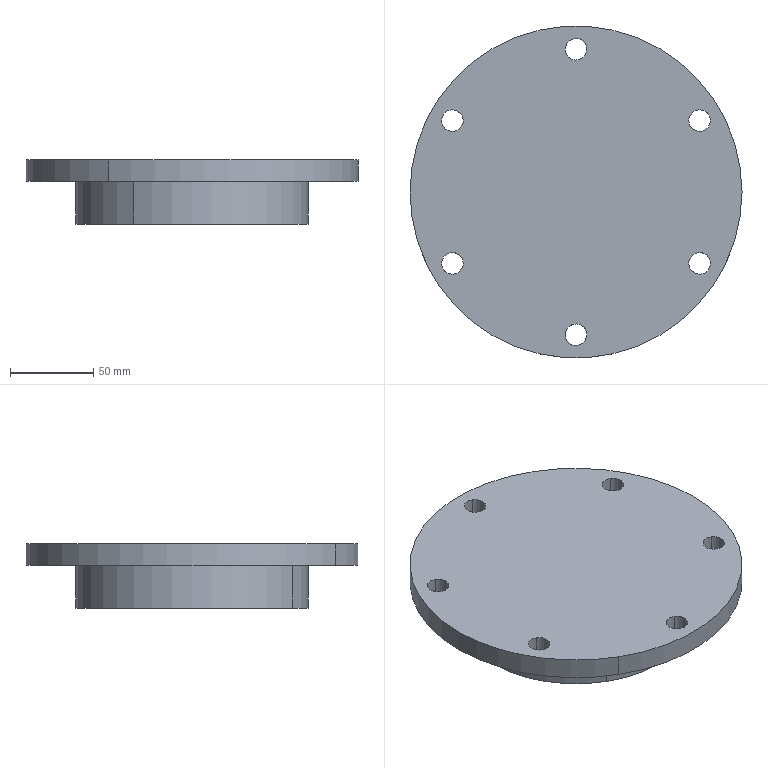Component | SolidWorks | PartAssemblyInLowerHousing-1_FlangeOnLowSpeedAxis1-1 | 1 solid | 22 faces | box 200 x 200 x 38.75 mm | volume 478948 mm3 | cylinder 16 | plane 4 | cone 2 | commonest cylinder face diameters 13 x12 200 x2 140 x2
build123d program:
from build123d import *

# Parameters (mm, degrees)
SKETCH2_R          = 6.5
CUT_EXTRUDE2_DEPTH = 147.634
CIRPATTERN1_COUNT  = 6
DRAFT1_ANGLE       = 2


with BuildPart() as part:
    # Sketch1 → Revolve1 (revolve)
    with BuildSketch(Plane.XY, mode=Mode.PRIVATE) as revolve1_sk:
        Polygon((0, 0), (13, 0), (13, 62), (38.75, 62), (38.75, 70), (13, 70), (13, 100), (0, 100), align=None)
    revolve(revolve1_sk.sketch.rotate(Axis((0, 0, 0), (1, 0, 0)), 90), axis=Axis((0, 0, 0), (1, 0, 0)))

    # Sketch2 → Cut-Extrude2 (cut, through all)
    with BuildSketch(Plane.ZY):
        with Locations((0, 86)):
            Circle(SKETCH2_R)
    cut_extrude2 = extrude(amount=-CUT_EXTRUDE2_DEPTH, mode=Mode.SUBTRACT)

    # CirPattern1: Cut-Extrude2 ×6 about axis
    cirpattern1_axis = Axis((0, 0, 0), (1, 0, 0))
    for i in range(1, CIRPATTERN1_COUNT):
        add(cut_extrude2.rotate(cirpattern1_axis, i * 360 / CIRPATTERN1_COUNT), mode=Mode.SUBTRACT)

    # Draft1
    draft1_faces = [part.faces().sort_by_distance(p)[0] for p in [
        (25.875, 0, -62),
    ]]
    draft(draft1_faces, Plane(origin=(13, 0, 0), x_dir=(0, 0, 1), z_dir=(1, 0, 0)), DRAFT1_ANGLE)


solid = part.part

# Placed as in the assembly
solid = solid.moved(Location((1140.83, 1268.591, 1836.217), (0, 90, 0)))
STEP:
#1=COLOUR_RGB('',0.7922,0.8196,0.9333);
#2=FILL_AREA_STYLE_COLOUR('',#1);
#3=FILL_AREA_STYLE('',(#2));
#4=SURFACE_STYLE_FILL_AREA(#3);
#5=SURFACE_SIDE_STYLE('',(#4));
#6=SURFACE_STYLE_USAGE(.BOTH.,#5);
#7=PRESENTATION_STYLE_ASSIGNMENT((#6));
#8=CARTESIAN_POINT('',(44.787,53.109,71.78));
#9=VERTEX_POINT('',#8);
#10=CARTESIAN_POINT('',(45.043,53.552,71.78));
#11=VERTEX_POINT('',#10);
#12=CARTESIAN_POINT('',(44.915,53.33,71.78));
#13=DIRECTION('',(0.,0.,1.));
#14=DIRECTION('',(0.5,0.866,0.));
#15=AXIS2_PLACEMENT_3D('',#12,#13,#14);
#16=CIRCLE('',#15,0.2559);
#17=EDGE_CURVE('',#9,#11,#16,.T.);
#18=ORIENTED_EDGE('',*,*,#17,.F.);
#19=CARTESIAN_POINT('',(44.787,53.109,72.292));
#20=VERTEX_POINT('',#19);
#21=CARTESIAN_POINT('',(44.787,53.109,70.766));
#22=DIRECTION('',(0.,0.,1.));
#23=VECTOR('',#22,39.37);
#24=LINE('',#21,#23);
#25=EDGE_CURVE('',#9,#20,#24,.T.);
#26=ORIENTED_EDGE('',*,*,#25,.T.);
#27=CARTESIAN_POINT('',(45.043,53.552,72.292));
#28=VERTEX_POINT('',#27);
#29=CARTESIAN_POINT('',(44.915,53.33,72.292));
#30=DIRECTION('',(0.,0.,1.));
#31=DIRECTION('',(1.,0.,0.));
#32=AXIS2_PLACEMENT_3D('',#29,#30,#31);
#33=CIRCLE('',#32,0.2559);
#34=EDGE_CURVE('',#20,#28,#33,.T.);
#35=ORIENTED_EDGE('',*,*,#34,.T.);
#36=CARTESIAN_POINT('',(45.043,53.552,70.766));
#37=DIRECTION('',(0.,0.,1.));
#38=VECTOR('',#37,39.37);
#39=LINE('',#36,#38);
#40=EDGE_CURVE('',#11,#28,#39,.T.);
#41=ORIENTED_EDGE('',*,*,#40,.F.);
#42=EDGE_LOOP('',(#18,#26,#35,#41));
#43=FACE_OUTER_BOUND('',#42,.T.);
#44=CARTESIAN_POINT('',(44.915,53.33,70.766));
#45=DIRECTION('',(0.,0.,1.));
#46=DIRECTION('',(0.5,0.866,0.));
#47=AXIS2_PLACEMENT_3D('',#44,#45,#46);
#48=CYLINDRICAL_SURFACE('',#47,0.2559);
#49=ADVANCED_FACE('',(#43),#48,.F.);
#50=CARTESIAN_POINT('',(47.719,51.416,71.78));
#51=VERTEX_POINT('',#50);
#52=CARTESIAN_POINT('',(47.975,51.859,71.78));
#53=VERTEX_POINT('',#52);
#54=CARTESIAN_POINT('',(47.847,51.637,71.78));
#55=DIRECTION('',(0.,0.,1.));
#56=DIRECTION('',(0.5,0.866,0.));
#57=AXIS2_PLACEMENT_3D('',#54,#55,#56);
#58=CIRCLE('',#57,0.2559);
#59=EDGE_CURVE('',#51,#53,#58,.T.);
#60=ORIENTED_EDGE('',*,*,#59,.F.);
#61=CARTESIAN_POINT('',(47.719,51.416,72.292));
#62=VERTEX_POINT('',#61);
#63=CARTESIAN_POINT('',(47.719,51.416,70.766));
#64=DIRECTION('',(0.,0.,1.));
#65=VECTOR('',#64,39.37);
#66=LINE('',#63,#65);
#67=EDGE_CURVE('',#51,#62,#66,.T.);
#68=ORIENTED_EDGE('',*,*,#67,.T.);
#69=CARTESIAN_POINT('',(47.975,51.859,72.292));
#70=VERTEX_POINT('',#69);
#71=CARTESIAN_POINT('',(47.847,51.637,72.292));
#72=DIRECTION('',(0.,0.,1.));
#73=DIRECTION('',(0.5,-0.866,0.));
#74=AXIS2_PLACEMENT_3D('',#71,#72,#73);
#75=CIRCLE('',#74,0.2559);
#76=EDGE_CURVE('',#62,#70,#75,.T.);
#77=ORIENTED_EDGE('',*,*,#76,.T.);
#78=CARTESIAN_POINT('',(47.975,51.859,70.766));
#79=DIRECTION('',(0.,0.,1.));
#80=VECTOR('',#79,39.37);
#81=LINE('',#78,#80);
#82=EDGE_CURVE('',#53,#70,#81,.T.);
#83=ORIENTED_EDGE('',*,*,#82,.F.);
#84=EDGE_LOOP('',(#60,#68,#77,#83));
#85=FACE_OUTER_BOUND('',#84,.T.);
#86=CARTESIAN_POINT('',(47.847,51.637,70.766));
#87=DIRECTION('',(0.,0.,1.));
#88=DIRECTION('',(0.5,0.866,0.));
#89=AXIS2_PLACEMENT_3D('',#86,#87,#88);
#90=CYLINDRICAL_SURFACE('',#89,0.2559);
#91=ADVANCED_FACE('',(#85),#90,.F.);
#92=CARTESIAN_POINT('',(47.719,48.03,71.78));
#93=VERTEX_POINT('',#92);
#94=CARTESIAN_POINT('',(47.975,48.473,71.78));
#95=VERTEX_POINT('',#94);
#96=CARTESIAN_POINT('',(47.847,48.252,71.78));
#97=DIRECTION('',(0.,0.,1.));
#98=DIRECTION('',(0.5,0.866,0.));
#99=AXIS2_PLACEMENT_3D('',#96,#97,#98);
#100=CIRCLE('',#99,0.2559);
#101=EDGE_CURVE('',#93,#95,#100,.T.);
#102=ORIENTED_EDGE('',*,*,#101,.F.);
#103=CARTESIAN_POINT('',(47.719,48.03,72.292));
#104=VERTEX_POINT('',#103);
#105=CARTESIAN_POINT('',(47.719,48.03,70.766));
#106=DIRECTION('',(0.,0.,1.));
#107=VECTOR('',#106,39.37);
#108=LINE('',#105,#107);
#109=EDGE_CURVE('',#93,#104,#108,.T.);
#110=ORIENTED_EDGE('',*,*,#109,.T.);
#111=CARTESIAN_POINT('',(47.975,48.473,72.292));
#112=VERTEX_POINT('',#111);
#113=CARTESIAN_POINT('',(47.847,48.252,72.292));
#114=DIRECTION('',(0.,0.,1.));
#115=DIRECTION('',(-0.5,-0.866,0.));
#116=AXIS2_PLACEMENT_3D('',#113,#114,#115);
#117=CIRCLE('',#116,0.2559);
#118=EDGE_CURVE('',#104,#112,#117,.T.);
#119=ORIENTED_EDGE('',*,*,#118,.T.);
#120=CARTESIAN_POINT('',(47.975,48.473,70.766));
#121=DIRECTION('',(0.,0.,1.));
#122=VECTOR('',#121,39.37);
#123=LINE('',#120,#122);
#124=EDGE_CURVE('',#95,#112,#123,.T.);
#125=ORIENTED_EDGE('',*,*,#124,.F.);
#126=EDGE_LOOP('',(#102,#110,#119,#125));
#127=FACE_OUTER_BOUND('',#126,.T.);
#128=CARTESIAN_POINT('',(47.847,48.252,70.766));
#129=DIRECTION('',(0.,0.,1.));
#130=DIRECTION('',(0.5,0.866,0.));
#131=AXIS2_PLACEMENT_3D('',#128,#129,#130);
#132=CYLINDRICAL_SURFACE('',#131,0.2559);
#133=ADVANCED_FACE('',(#127),#132,.F.);
#134=CARTESIAN_POINT('',(44.787,46.337,71.78));
#135=VERTEX_POINT('',#134);
#136=CARTESIAN_POINT('',(45.043,46.78,71.78));
#137=VERTEX_POINT('',#136);
#138=CARTESIAN_POINT('',(44.915,46.559,71.78));
#139=DIRECTION('',(0.,0.,1.));
#140=DIRECTION('',(0.5,0.866,0.));
#141=AXIS2_PLACEMENT_3D('',#138,#139,#140);
#142=CIRCLE('',#141,0.2559);
#143=EDGE_CURVE('',#135,#137,#142,.T.);
#144=ORIENTED_EDGE('',*,*,#143,.F.);
#145=CARTESIAN_POINT('',(44.787,46.337,72.292));
#146=VERTEX_POINT('',#145);
#147=CARTESIAN_POINT('',(44.787,46.337,70.766));
#148=DIRECTION('',(0.,0.,1.));
#149=VECTOR('',#148,39.37);
#150=LINE('',#147,#149);
#151=EDGE_CURVE('',#135,#146,#150,.T.);
#152=ORIENTED_EDGE('',*,*,#151,.T.);
#153=CARTESIAN_POINT('',(45.043,46.78,72.292));
#154=VERTEX_POINT('',#153);
#155=CARTESIAN_POINT('',(44.915,46.559,72.292));
#156=DIRECTION('',(0.,0.,1.));
#157=DIRECTION('',(-1.,0.,0.));
#158=AXIS2_PLACEMENT_3D('',#155,#156,#157);
#159=CIRCLE('',#158,0.2559);
#160=EDGE_CURVE('',#146,#154,#159,.T.);
#161=ORIENTED_EDGE('',*,*,#160,.T.);
#162=CARTESIAN_POINT('',(45.043,46.78,70.766));
#163=DIRECTION('',(0.,0.,1.));
#164=VECTOR('',#163,39.37);
#165=LINE('',#162,#164);
#166=EDGE_CURVE('',#137,#154,#165,.T.);
#167=ORIENTED_EDGE('',*,*,#166,.F.);
#168=EDGE_LOOP('',(#144,#152,#161,#167));
#169=FACE_OUTER_BOUND('',#168,.T.);
#170=CARTESIAN_POINT('',(44.915,46.559,70.766));
#171=DIRECTION('',(0.,0.,1.));
#172=DIRECTION('',(0.5,0.866,0.));
#173=AXIS2_PLACEMENT_3D('',#170,#171,#172);
#174=CYLINDRICAL_SURFACE('',#173,0.2559);
#175=ADVANCED_FACE('',(#169),#174,.F.);
#176=CARTESIAN_POINT('',(41.854,48.03,71.78));
#177=VERTEX_POINT('',#176);
#178=CARTESIAN_POINT('',(42.11,48.473,71.78));
#179=VERTEX_POINT('',#178);
#180=CARTESIAN_POINT('',(41.982,48.252,71.78));
#181=DIRECTION('',(0.,0.,1.));
#182=DIRECTION('',(0.5,0.866,0.));
#183=AXIS2_PLACEMENT_3D('',#180,#181,#182);
#184=CIRCLE('',#183,0.2559);
#185=EDGE_CURVE('',#177,#179,#184,.T.);
#186=ORIENTED_EDGE('',*,*,#185,.F.);
#187=CARTESIAN_POINT('',(41.854,48.03,72.292));
#188=VERTEX_POINT('',#187);
#189=CARTESIAN_POINT('',(41.854,48.03,70.766));
#190=DIRECTION('',(0.,0.,1.));
#191=VECTOR('',#190,39.37);
#192=LINE('',#189,#191);
#193=EDGE_CURVE('',#177,#188,#192,.T.);
#194=ORIENTED_EDGE('',*,*,#193,.T.);
#195=CARTESIAN_POINT('',(42.11,48.473,72.292));
#196=VERTEX_POINT('',#195);
#197=CARTESIAN_POINT('',(41.982,48.252,72.292));
#198=DIRECTION('',(0.,0.,1.));
#199=DIRECTION('',(-0.5,0.866,0.));
#200=AXIS2_PLACEMENT_3D('',#197,#198,#199);
#201=CIRCLE('',#200,0.2559);
#202=EDGE_CURVE('',#188,#196,#201,.T.);
#203=ORIENTED_EDGE('',*,*,#202,.T.);
#204=CARTESIAN_POINT('',(42.11,48.473,70.766));
#205=DIRECTION('',(0.,0.,1.));
#206=VECTOR('',#205,39.37);
#207=LINE('',#204,#206);
#208=EDGE_CURVE('',#179,#196,#207,.T.);
#209=ORIENTED_EDGE('',*,*,#208,.F.);
#210=EDGE_LOOP('',(#186,#194,#203,#209));
#211=FACE_OUTER_BOUND('',#210,.T.);
#212=CARTESIAN_POINT('',(41.982,48.252,70.766));
#213=DIRECTION('',(0.,0.,1.));
#214=DIRECTION('',(0.5,0.866,0.));
#215=AXIS2_PLACEMENT_3D('',#212,#213,#214);
#216=CYLINDRICAL_SURFACE('',#215,0.2559);
#217=ADVANCED_FACE('',(#211),#216,.F.);
#218=CARTESIAN_POINT('',(41.854,51.416,71.78));
#219=VERTEX_POINT('',#218);
#220=CARTESIAN_POINT('',(42.11,51.859,71.78));
#221=VERTEX_POINT('',#220);
#222=CARTESIAN_POINT('',(41.982,51.637,71.78));
#223=DIRECTION('',(0.,0.,1.));
#224=DIRECTION('',(0.5,0.866,0.));
#225=AXIS2_PLACEMENT_3D('',#222,#223,#224);
#226=CIRCLE('',#225,0.2559);
#227=EDGE_CURVE('',#219,#221,#226,.T.);
#228=ORIENTED_EDGE('',*,*,#227,.F.);
#229=CARTESIAN_POINT('',(41.854,51.416,72.292));
#230=VERTEX_POINT('',#229);
#231=CARTESIAN_POINT('',(41.854,51.416,70.766));
#232=DIRECTION('',(0.,0.,1.));
#233=VECTOR('',#232,39.37);
#234=LINE('',#231,#233);
#235=EDGE_CURVE('',#219,#230,#234,.T.);
#236=ORIENTED_EDGE('',*,*,#235,.T.);
#237=CARTESIAN_POINT('',(42.11,51.859,72.292));
#238=VERTEX_POINT('',#237);
#239=CARTESIAN_POINT('',(41.982,51.637,72.292));
#240=DIRECTION('',(0.,0.,1.));
#241=DIRECTION('',(0.5,0.866,0.));
#242=AXIS2_PLACEMENT_3D('',#239,#240,#241);
#243=CIRCLE('',#242,0.2559);
#244=EDGE_CURVE('',#230,#238,#243,.T.);
#245=ORIENTED_EDGE('',*,*,#244,.T.);
#246=CARTESIAN_POINT('',(42.11,51.859,70.766));
#247=DIRECTION('',(0.,0.,1.));
#248=VECTOR('',#247,39.37);
#249=LINE('',#246,#248);
#250=EDGE_CURVE('',#221,#238,#249,.T.);
#251=ORIENTED_EDGE('',*,*,#250,.F.);
#252=EDGE_LOOP('',(#228,#236,#245,#251));
#253=FACE_OUTER_BOUND('',#252,.T.);
#254=CARTESIAN_POINT('',(41.982,51.637,70.766));
#255=DIRECTION('',(0.,0.,1.));
#256=DIRECTION('',(0.5,0.866,0.));
#257=AXIS2_PLACEMENT_3D('',#254,#255,#256);
#258=CYLINDRICAL_SURFACE('',#257,0.2559);
#259=ADVANCED_FACE('',(#253),#258,.F.);
#260=CARTESIAN_POINT('',(46.883,53.354,71.78));
#261=VERTEX_POINT('',#260);
#262=CARTESIAN_POINT('',(42.946,46.535,71.78));
#263=VERTEX_POINT('',#262);
#264=CARTESIAN_POINT('',(44.915,49.945,71.78));
#265=DIRECTION('',(0.,0.,1.));
#266=DIRECTION('',(0.5,0.866,0.));
#267=AXIS2_PLACEMENT_3D('',#264,#265,#266);
#268=CIRCLE('',#267,3.937);
#269=EDGE_CURVE('',#261,#263,#268,.T.);
#270=ORIENTED_EDGE('',*,*,#269,.T.);
#271=CARTESIAN_POINT('',(42.946,46.535,72.292));
#272=VERTEX_POINT('',#271);
#273=CARTESIAN_POINT('',(42.946,46.535,72.292));
#274=DIRECTION('',(0.,0.,1.));
#275=VECTOR('',#274,39.37);
#276=LINE('',#273,#275);
#277=EDGE_CURVE('',#263,#272,#276,.T.);
#278=ORIENTED_EDGE('',*,*,#277,.T.);
#279=CARTESIAN_POINT('',(46.883,53.354,72.292));
#280=VERTEX_POINT('',#279);
#281=CARTESIAN_POINT('',(44.915,49.945,72.292));
#282=DIRECTION('',(0.,0.,1.));
#283=DIRECTION('',(0.5,0.866,0.));
#284=AXIS2_PLACEMENT_3D('',#281,#282,#283);
#285=CIRCLE('',#284,3.937);
#286=EDGE_CURVE('',#280,#272,#285,.T.);
#287=ORIENTED_EDGE('',*,*,#286,.F.);
#288=CARTESIAN_POINT('',(46.883,53.354,72.292));
#289=DIRECTION('',(0.,0.,1.));
#290=VECTOR('',#289,39.37);
#291=LINE('',#288,#290);
#292=EDGE_CURVE('',#261,#280,#291,.T.);
#293=ORIENTED_EDGE('',*,*,#292,.F.);
#294=EDGE_LOOP('',(#270,#278,#287,#293));
#295=FACE_OUTER_BOUND('',#294,.T.);
#296=CARTESIAN_POINT('',(44.915,49.945,72.292));
#297=DIRECTION('',(0.,0.,1.));
#298=DIRECTION('',(0.5,0.866,0.));
#299=AXIS2_PLACEMENT_3D('',#296,#297,#298);
#300=CYLINDRICAL_SURFACE('',#299,3.937);
#301=ADVANCED_FACE('',(#295),#300,.T.);
#302=CARTESIAN_POINT('',(46.293,52.331,70.766));
#303=VERTEX_POINT('',#302);
#304=CARTESIAN_POINT('',(43.537,47.558,70.766));
#305=VERTEX_POINT('',#304);
#306=CARTESIAN_POINT('',(44.915,49.945,70.766));
#307=DIRECTION('',(0.,0.,1.));
#308=DIRECTION('',(0.5,0.866,0.));
#309=AXIS2_PLACEMENT_3D('',#306,#307,#308);
#310=CIRCLE('',#309,2.756);
#311=EDGE_CURVE('',#303,#305,#310,.T.);
#312=ORIENTED_EDGE('',*,*,#311,.T.);
#313=CARTESIAN_POINT('',(43.537,47.558,71.78));
#314=VERTEX_POINT('',#313);
#315=CARTESIAN_POINT('',(43.537,47.558,72.292));
#316=DIRECTION('',(0.,0.,1.));
#317=VECTOR('',#316,39.37);
#318=LINE('',#315,#317);
#319=EDGE_CURVE('',#305,#314,#318,.T.);
#320=ORIENTED_EDGE('',*,*,#319,.T.);
#321=CARTESIAN_POINT('',(46.293,52.331,71.78));
#322=VERTEX_POINT('',#321);
#323=CARTESIAN_POINT('',(44.915,49.945,71.78));
#324=DIRECTION('',(0.,0.,1.));
#325=DIRECTION('',(0.5,0.866,0.));
#326=AXIS2_PLACEMENT_3D('',#323,#324,#325);
#327=CIRCLE('',#326,2.756);
#328=EDGE_CURVE('',#322,#314,#327,.T.);
#329=ORIENTED_EDGE('',*,*,#328,.F.);
#330=CARTESIAN_POINT('',(46.293,52.331,72.292));
#331=DIRECTION('',(0.,0.,1.));
#332=VECTOR('',#331,39.37);
#333=LINE('',#330,#332);
#334=EDGE_CURVE('',#303,#322,#333,.T.);
#335=ORIENTED_EDGE('',*,*,#334,.F.);
#336=EDGE_LOOP('',(#312,#320,#329,#335));
#337=FACE_OUTER_BOUND('',#336,.T.);
#338=CARTESIAN_POINT('',(44.915,49.945,72.292));
#339=DIRECTION('',(0.,0.,1.));
#340=DIRECTION('',(0.5,0.866,0.));
#341=AXIS2_PLACEMENT_3D('',#338,#339,#340);
#342=CYLINDRICAL_SURFACE('',#341,2.756);
#343=ADVANCED_FACE('',(#337),#342,.T.);
#344=CARTESIAN_POINT('',(46.135,52.058,71.78));
#345=VERTEX_POINT('',#344);
#346=CARTESIAN_POINT('',(43.694,47.831,71.78));
#347=VERTEX_POINT('',#346);
#348=CARTESIAN_POINT('',(44.915,49.945,71.78));
#349=DIRECTION('',(0.,0.,1.));
#350=DIRECTION('',(0.5,0.866,0.));
#351=AXIS2_PLACEMENT_3D('',#348,#349,#350);
#352=CIRCLE('',#351,2.441);
#353=EDGE_CURVE('',#345,#347,#352,.T.);
#354=ORIENTED_EDGE('',*,*,#353,.T.);
#355=CARTESIAN_POINT('',(43.676,47.8,70.766));
#356=VERTEX_POINT('',#355);
#357=CARTESIAN_POINT('',(43.694,47.831,71.78));
#358=DIRECTION('',(-0.01745,-0.03022,-0.9994));
#359=VECTOR('',#358,39.37);
#360=LINE('',#357,#359);
#361=EDGE_CURVE('',#347,#356,#360,.T.);
#362=ORIENTED_EDGE('',*,*,#361,.T.);
#363=CARTESIAN_POINT('',(46.153,52.089,70.766));
#364=VERTEX_POINT('',#363);
#365=CARTESIAN_POINT('',(44.915,49.945,70.766));
#366=DIRECTION('',(0.,0.,1.));
#367=DIRECTION('',(0.5,0.866,0.));
#368=AXIS2_PLACEMENT_3D('',#365,#366,#367);
#369=CIRCLE('',#368,2.476);
#370=EDGE_CURVE('',#364,#356,#369,.T.);
#371=ORIENTED_EDGE('',*,*,#370,.F.);
#372=CARTESIAN_POINT('',(46.135,52.058,71.78));
#373=DIRECTION('',(0.01745,0.03022,-0.9994));
#374=VECTOR('',#373,39.37);
#375=LINE('',#372,#374);
#376=EDGE_CURVE('',#345,#364,#375,.T.);
#377=ORIENTED_EDGE('',*,*,#376,.F.);
#378=EDGE_LOOP('',(#354,#362,#371,#377));
#379=FACE_OUTER_BOUND('',#378,.T.);
#380=CARTESIAN_POINT('',(44.915,49.945,71.78));
#381=DIRECTION('',(0.,0.,-1.));
#382=DIRECTION('',(0.5,0.866,0.));
#383=AXIS2_PLACEMENT_3D('',#380,#381,#382);
#384=CONICAL_SURFACE('',#383,2.441,0.03491);
#385=ADVANCED_FACE('',(#379),#384,.F.);
#386=CARTESIAN_POINT('',(44.915,53.33,72.292));
#387=DIRECTION('',(0.,0.,1.));
#388=DIRECTION('',(1.,0.,0.));
#389=AXIS2_PLACEMENT_3D('',#386,#387,#388);
#390=CIRCLE('',#389,0.2559);
#391=EDGE_CURVE('',#28,#20,#390,.T.);
#392=ORIENTED_EDGE('',*,*,#391,.F.);
#393=ORIENTED_EDGE('',*,*,#34,.F.);
#394=EDGE_LOOP('',(#392,#393));
#395=FACE_BOUND('',#394,.T.);
#396=CARTESIAN_POINT('',(47.847,51.637,72.292));
#397=DIRECTION('',(0.,0.,1.));
#398=DIRECTION('',(0.5,-0.866,0.));
#399=AXIS2_PLACEMENT_3D('',#396,#397,#398);
#400=CIRCLE('',#399,0.2559);
#401=EDGE_CURVE('',#70,#62,#400,.T.);
#402=ORIENTED_EDGE('',*,*,#401,.F.);
#403=ORIENTED_EDGE('',*,*,#76,.F.);
#404=EDGE_LOOP('',(#402,#403));
#405=FACE_BOUND('',#404,.T.);
#406=CARTESIAN_POINT('',(47.847,48.252,72.292));
#407=DIRECTION('',(0.,0.,1.));
#408=DIRECTION('',(-0.5,-0.866,0.));
#409=AXIS2_PLACEMENT_3D('',#406,#407,#408);
#410=CIRCLE('',#409,0.2559);
#411=EDGE_CURVE('',#112,#104,#410,.T.);
#412=ORIENTED_EDGE('',*,*,#411,.F.);
#413=ORIENTED_EDGE('',*,*,#118,.F.);
#414=EDGE_LOOP('',(#412,#413));
#415=FACE_BOUND('',#414,.T.);
#416=CARTESIAN_POINT('',(44.915,46.559,72.292));
#417=DIRECTION('',(0.,0.,1.));
#418=DIRECTION('',(-1.,0.,0.));
#419=AXIS2_PLACEMENT_3D('',#416,#417,#418);
#420=CIRCLE('',#419,0.2559);
#421=EDGE_CURVE('',#154,#146,#420,.T.);
#422=ORIENTED_EDGE('',*,*,#421,.F.);
#423=ORIENTED_EDGE('',*,*,#160,.F.);
#424=EDGE_LOOP('',(#422,#423));
#425=FACE_BOUND('',#424,.T.);
#426=CARTESIAN_POINT('',(41.982,48.252,72.292));
#427=DIRECTION('',(0.,0.,1.));
#428=DIRECTION('',(-0.5,0.866,0.));
#429=AXIS2_PLACEMENT_3D('',#426,#427,#428);
#430=CIRCLE('',#429,0.2559);
#431=EDGE_CURVE('',#196,#188,#430,.T.);
#432=ORIENTED_EDGE('',*,*,#431,.F.);
#433=ORIENTED_EDGE('',*,*,#202,.F.);
#434=EDGE_LOOP('',(#432,#433));
#435=FACE_BOUND('',#434,.T.);
#436=CARTESIAN_POINT('',(41.982,51.637,72.292));
#437=DIRECTION('',(0.,0.,1.));
#438=DIRECTION('',(0.5,0.866,0.));
#439=AXIS2_PLACEMENT_3D('',#436,#437,#438);
#440=CIRCLE('',#439,0.2559);
#441=EDGE_CURVE('',#238,#230,#440,.T.);
#442=ORIENTED_EDGE('',*,*,#441,.F.);
#443=ORIENTED_EDGE('',*,*,#244,.F.);
#444=EDGE_LOOP('',(#442,#443));
#445=FACE_BOUND('',#444,.T.);
#446=ORIENTED_EDGE('',*,*,#286,.T.);
#447=CARTESIAN_POINT('',(44.915,49.945,72.292));
#448=DIRECTION('',(0.,0.,1.));
#449=DIRECTION('',(0.5,0.866,0.));
#450=AXIS2_PLACEMENT_3D('',#447,#448,#449);
#451=CIRCLE('',#450,3.937);
#452=EDGE_CURVE('',#272,#280,#451,.T.);
#453=ORIENTED_EDGE('',*,*,#452,.T.);
#454=EDGE_LOOP('',(#446,#453));
#455=FACE_OUTER_BOUND('',#454,.T.);
#456=CARTESIAN_POINT('',(41.505,51.913,72.292));
#457=DIRECTION('',(0.,0.,-1.));
#458=DIRECTION('',(-0.5,-0.866,0.));
#459=AXIS2_PLACEMENT_3D('',#456,#457,#458);
#460=PLANE('',#459);
#461=ADVANCED_FACE('',(#395,#405,#415,#425,#435,#445,#455),#460,.F.);
#462=ORIENTED_EDGE('',*,*,#353,.F.);
#463=CARTESIAN_POINT('',(44.915,49.945,71.78));
#464=DIRECTION('',(0.,0.,1.));
#465=DIRECTION('',(0.5,0.866,0.));
#466=AXIS2_PLACEMENT_3D('',#463,#464,#465);
#467=CIRCLE('',#466,2.441);
#468=EDGE_CURVE('',#347,#345,#467,.T.);
#469=ORIENTED_EDGE('',*,*,#468,.F.);
#470=EDGE_LOOP('',(#462,#469));
#471=FACE_OUTER_BOUND('',#470,.T.);
#472=CARTESIAN_POINT('',(44.915,49.945,71.78));
#473=DIRECTION('',(0.,0.,1.));
#474=DIRECTION('',(0.5,0.866,0.));
#475=AXIS2_PLACEMENT_3D('',#472,#473,#474);
#476=PLANE('',#475);
#477=ADVANCED_FACE('',(#471),#476,.F.);
#478=ORIENTED_EDGE('',*,*,#361,.F.);
#479=ORIENTED_EDGE('',*,*,#468,.T.);
#480=ORIENTED_EDGE('',*,*,#376,.T.);
#481=CARTESIAN_POINT('',(44.915,49.945,70.766));
#482=DIRECTION('',(0.,0.,1.));
#483=DIRECTION('',(0.5,0.866,0.));
#484=AXIS2_PLACEMENT_3D('',#481,#482,#483);
#485=CIRCLE('',#484,2.476);
#486=EDGE_CURVE('',#356,#364,#485,.T.);
#487=ORIENTED_EDGE('',*,*,#486,.F.);
#488=EDGE_LOOP('',(#478,#479,#480,#487));
#489=FACE_OUTER_BOUND('',#488,.T.);
#490=CARTESIAN_POINT('',(44.915,49.945,71.78));
#491=DIRECTION('',(0.,0.,-1.));
#492=DIRECTION('',(0.5,0.866,0.));
#493=AXIS2_PLACEMENT_3D('',#490,#491,#492);
#494=CONICAL_SURFACE('',#493,2.441,0.03491);
#495=ADVANCED_FACE('',(#489),#494,.F.);
#496=ORIENTED_EDGE('',*,*,#311,.F.);
#497=CARTESIAN_POINT('',(44.915,49.945,70.766));
#498=DIRECTION('',(0.,0.,1.));
#499=DIRECTION('',(0.5,0.866,0.));
#500=AXIS2_PLACEMENT_3D('',#497,#498,#499);
#501=CIRCLE('',#500,2.756);
#502=EDGE_CURVE('',#305,#303,#501,.T.);
#503=ORIENTED_EDGE('',*,*,#502,.F.);
#504=EDGE_LOOP('',(#496,#503));
#505=FACE_OUTER_BOUND('',#504,.T.);
#506=ORIENTED_EDGE('',*,*,#370,.T.);
#507=ORIENTED_EDGE('',*,*,#486,.T.);
#508=EDGE_LOOP('',(#506,#507));
#509=FACE_BOUND('',#508,.T.);
#510=CARTESIAN_POINT('',(42.801,51.165,70.766));
#511=DIRECTION('',(0.,0.,1.));
#512=DIRECTION('',(0.5,0.866,0.));
#513=AXIS2_PLACEMENT_3D('',#510,#511,#512);
#514=PLANE('',#513);
#515=ADVANCED_FACE('',(#505,#509),#514,.F.);
#516=ORIENTED_EDGE('',*,*,#319,.F.);
#517=ORIENTED_EDGE('',*,*,#502,.T.);
#518=ORIENTED_EDGE('',*,*,#334,.T.);
#519=CARTESIAN_POINT('',(44.915,49.945,71.78));
#520=DIRECTION('',(0.,0.,1.));
#521=DIRECTION('',(0.5,0.866,0.));
#522=AXIS2_PLACEMENT_3D('',#519,#520,#521);
#523=CIRCLE('',#522,2.756);
#524=EDGE_CURVE('',#314,#322,#523,.T.);
#525=ORIENTED_EDGE('',*,*,#524,.F.);
#526=EDGE_LOOP('',(#516,#517,#518,#525));
#527=FACE_OUTER_BOUND('',#526,.T.);
#528=CARTESIAN_POINT('',(44.915,49.945,72.292));
#529=DIRECTION('',(0.,0.,1.));
#530=DIRECTION('',(0.5,0.866,0.));
#531=AXIS2_PLACEMENT_3D('',#528,#529,#530);
#532=CYLINDRICAL_SURFACE('',#531,2.756);
#533=ADVANCED_FACE('',(#527),#532,.T.);
#534=CARTESIAN_POINT('',(44.915,53.33,71.78));
#535=DIRECTION('',(0.,0.,1.));
#536=DIRECTION('',(0.5,0.866,0.));
#537=AXIS2_PLACEMENT_3D('',#534,#535,#536);
#538=CIRCLE('',#537,0.2559);
#539=EDGE_CURVE('',#11,#9,#538,.T.);
#540=ORIENTED_EDGE('',*,*,#539,.T.);
#541=ORIENTED_EDGE('',*,*,#17,.T.);
#542=EDGE_LOOP('',(#540,#541));
#543=FACE_BOUND('',#542,.T.);
#544=CARTESIAN_POINT('',(47.847,51.637,71.78));
#545=DIRECTION('',(0.,0.,1.));
#546=DIRECTION('',(0.5,0.866,0.));
#547=AXIS2_PLACEMENT_3D('',#544,#545,#546);
#548=CIRCLE('',#547,0.2559);
#549=EDGE_CURVE('',#53,#51,#548,.T.);
#550=ORIENTED_EDGE('',*,*,#549,.T.);
#551=ORIENTED_EDGE('',*,*,#59,.T.);
#552=EDGE_LOOP('',(#550,#551));
#553=FACE_BOUND('',#552,.T.);
#554=CARTESIAN_POINT('',(47.847,48.252,71.78));
#555=DIRECTION('',(0.,0.,1.));
#556=DIRECTION('',(0.5,0.866,0.));
#557=AXIS2_PLACEMENT_3D('',#554,#555,#556);
#558=CIRCLE('',#557,0.2559);
#559=EDGE_CURVE('',#95,#93,#558,.T.);
#560=ORIENTED_EDGE('',*,*,#559,.T.);
#561=ORIENTED_EDGE('',*,*,#101,.T.);
#562=EDGE_LOOP('',(#560,#561));
#563=FACE_BOUND('',#562,.T.);
#564=CARTESIAN_POINT('',(44.915,46.559,71.78));
#565=DIRECTION('',(0.,0.,1.));
#566=DIRECTION('',(0.5,0.866,0.));
#567=AXIS2_PLACEMENT_3D('',#564,#565,#566);
#568=CIRCLE('',#567,0.2559);
#569=EDGE_CURVE('',#137,#135,#568,.T.);
#570=ORIENTED_EDGE('',*,*,#569,.T.);
#571=ORIENTED_EDGE('',*,*,#143,.T.);
#572=EDGE_LOOP('',(#570,#571));
#573=FACE_BOUND('',#572,.T.);
#574=CARTESIAN_POINT('',(41.982,48.252,71.78));
#575=DIRECTION('',(0.,0.,1.));
#576=DIRECTION('',(0.5,0.866,0.));
#577=AXIS2_PLACEMENT_3D('',#574,#575,#576);
#578=CIRCLE('',#577,0.2559);
#579=EDGE_CURVE('',#179,#177,#578,.T.);
#580=ORIENTED_EDGE('',*,*,#579,.T.);
#581=ORIENTED_EDGE('',*,*,#185,.T.);
#582=EDGE_LOOP('',(#580,#581));
#583=FACE_BOUND('',#582,.T.);
#584=CARTESIAN_POINT('',(41.982,51.637,71.78));
#585=DIRECTION('',(0.,0.,1.));
#586=DIRECTION('',(0.5,0.866,0.));
#587=AXIS2_PLACEMENT_3D('',#584,#585,#586);
#588=CIRCLE('',#587,0.2559);
#589=EDGE_CURVE('',#221,#219,#588,.T.);
#590=ORIENTED_EDGE('',*,*,#589,.T.);
#591=ORIENTED_EDGE('',*,*,#227,.T.);
#592=EDGE_LOOP('',(#590,#591));
#593=FACE_BOUND('',#592,.T.);
#594=ORIENTED_EDGE('',*,*,#269,.F.);
#595=CARTESIAN_POINT('',(44.915,49.945,71.78));
#596=DIRECTION('',(0.,0.,1.));
#597=DIRECTION('',(0.5,0.866,0.));
#598=AXIS2_PLACEMENT_3D('',#595,#596,#597);
#599=CIRCLE('',#598,3.937);
#600=EDGE_CURVE('',#263,#261,#599,.T.);
#601=ORIENTED_EDGE('',*,*,#600,.F.);
#602=EDGE_LOOP('',(#594,#601));
#603=FACE_OUTER_BOUND('',#602,.T.);
#604=ORIENTED_EDGE('',*,*,#328,.T.);
#605=ORIENTED_EDGE('',*,*,#524,.T.);
#606=EDGE_LOOP('',(#604,#605));
#607=FACE_BOUND('',#606,.T.);
#608=CARTESIAN_POINT('',(42.528,51.322,71.78));
#609=DIRECTION('',(0.,0.,1.));
#610=DIRECTION('',(0.5,0.866,0.));
#611=AXIS2_PLACEMENT_3D('',#608,#609,#610);
#612=PLANE('',#611);
#613=ADVANCED_FACE('',(#543,#553,#563,#573,#583,#593,#603,#607),#612,.F.);
#614=ORIENTED_EDGE('',*,*,#277,.F.);
#615=ORIENTED_EDGE('',*,*,#600,.T.);
#616=ORIENTED_EDGE('',*,*,#292,.T.);
#617=ORIENTED_EDGE('',*,*,#452,.F.);
#618=EDGE_LOOP('',(#614,#615,#616,#617));
#619=FACE_OUTER_BOUND('',#618,.T.);
#620=CARTESIAN_POINT('',(44.915,49.945,72.292));
#621=DIRECTION('',(0.,0.,1.));
#622=DIRECTION('',(0.5,0.866,0.));
#623=AXIS2_PLACEMENT_3D('',#620,#621,#622);
#624=CYLINDRICAL_SURFACE('',#623,3.937);
#625=ADVANCED_FACE('',(#619),#624,.T.);
#626=ORIENTED_EDGE('',*,*,#235,.F.);
#627=ORIENTED_EDGE('',*,*,#589,.F.);
#628=ORIENTED_EDGE('',*,*,#250,.T.);
#629=ORIENTED_EDGE('',*,*,#441,.T.);
#630=EDGE_LOOP('',(#626,#627,#628,#629));
#631=FACE_OUTER_BOUND('',#630,.T.);
#632=CARTESIAN_POINT('',(41.982,51.637,70.766));
#633=DIRECTION('',(0.,0.,1.));
#634=DIRECTION('',(0.5,0.866,0.));
#635=AXIS2_PLACEMENT_3D('',#632,#633,#634);
#636=CYLINDRICAL_SURFACE('',#635,0.2559);
#637=ADVANCED_FACE('',(#631),#636,.F.);
#638=ORIENTED_EDGE('',*,*,#193,.F.);
#639=ORIENTED_EDGE('',*,*,#579,.F.);
#640=ORIENTED_EDGE('',*,*,#208,.T.);
#641=ORIENTED_EDGE('',*,*,#431,.T.);
#642=EDGE_LOOP('',(#638,#639,#640,#641));
#643=FACE_OUTER_BOUND('',#642,.T.);
#644=CARTESIAN_POINT('',(41.982,48.252,70.766));
#645=DIRECTION('',(0.,0.,1.));
#646=DIRECTION('',(0.5,0.866,0.));
#647=AXIS2_PLACEMENT_3D('',#644,#645,#646);
#648=CYLINDRICAL_SURFACE('',#647,0.2559);
#649=ADVANCED_FACE('',(#643),#648,.F.);
#650=ORIENTED_EDGE('',*,*,#151,.F.);
#651=ORIENTED_EDGE('',*,*,#569,.F.);
#652=ORIENTED_EDGE('',*,*,#166,.T.);
#653=ORIENTED_EDGE('',*,*,#421,.T.);
#654=EDGE_LOOP('',(#650,#651,#652,#653));
#655=FACE_OUTER_BOUND('',#654,.T.);
#656=CARTESIAN_POINT('',(44.915,46.559,70.766));
#657=DIRECTION('',(0.,0.,1.));
#658=DIRECTION('',(0.5,0.866,0.));
#659=AXIS2_PLACEMENT_3D('',#656,#657,#658);
#660=CYLINDRICAL_SURFACE('',#659,0.2559);
#661=ADVANCED_FACE('',(#655),#660,.F.);
#662=ORIENTED_EDGE('',*,*,#109,.F.);
#663=ORIENTED_EDGE('',*,*,#559,.F.);
#664=ORIENTED_EDGE('',*,*,#124,.T.);
#665=ORIENTED_EDGE('',*,*,#411,.T.);
#666=EDGE_LOOP('',(#662,#663,#664,#665));
#667=FACE_OUTER_BOUND('',#666,.T.);
#668=CARTESIAN_POINT('',(47.847,48.252,70.766));
#669=DIRECTION('',(0.,0.,1.));
#670=DIRECTION('',(0.5,0.866,0.));
#671=AXIS2_PLACEMENT_3D('',#668,#669,#670);
#672=CYLINDRICAL_SURFACE('',#671,0.2559);
#673=ADVANCED_FACE('',(#667),#672,.F.);
#674=ORIENTED_EDGE('',*,*,#67,.F.);
#675=ORIENTED_EDGE('',*,*,#549,.F.);
#676=ORIENTED_EDGE('',*,*,#82,.T.);
#677=ORIENTED_EDGE('',*,*,#401,.T.);
#678=EDGE_LOOP('',(#674,#675,#676,#677));
#679=FACE_OUTER_BOUND('',#678,.T.);
#680=CARTESIAN_POINT('',(47.847,51.637,70.766));
#681=DIRECTION('',(0.,0.,1.));
#682=DIRECTION('',(0.5,0.866,0.));
#683=AXIS2_PLACEMENT_3D('',#680,#681,#682);
#684=CYLINDRICAL_SURFACE('',#683,0.2559);
#685=ADVANCED_FACE('',(#679),#684,.F.);
#686=ORIENTED_EDGE('',*,*,#25,.F.);
#687=ORIENTED_EDGE('',*,*,#539,.F.);
#688=ORIENTED_EDGE('',*,*,#40,.T.);
#689=ORIENTED_EDGE('',*,*,#391,.T.);
#690=EDGE_LOOP('',(#686,#687,#688,#689));
#691=FACE_OUTER_BOUND('',#690,.T.);
#692=CARTESIAN_POINT('',(44.915,53.33,70.766));
#693=DIRECTION('',(0.,0.,1.));
#694=DIRECTION('',(0.5,0.866,0.));
#695=AXIS2_PLACEMENT_3D('',#692,#693,#694);
#696=CYLINDRICAL_SURFACE('',#695,0.2559);
#697=ADVANCED_FACE('',(#691),#696,.F.);
#698=CLOSED_SHELL('',(#49,#91,#133,#175,#217,#259,#301,#343,#385,#461,#477,#495,#515,#533,#613,#625,#637,#649,#661,#673,#685,#697));
#699=MANIFOLD_SOLID_BREP('',#698);
#700=STYLED_ITEM('',(#7),#699);
#701=(LENGTH_UNIT()NAMED_UNIT(*)SI_UNIT($,.METRE.));
#702=LENGTH_MEASURE_WITH_UNIT(LENGTH_MEASURE(0.0254),#701);
#703=DIMENSIONAL_EXPONENTS(1.,0.,0.,0.,0.,0.,0.);
#704=(CONVERSION_BASED_UNIT('',#702)LENGTH_UNIT()NAMED_UNIT(#703));
#705=UNCERTAINTY_MEASURE_WITH_UNIT(LENGTH_MEASURE(0.00001),#704,'','');
#706=(NAMED_UNIT(*)PLANE_ANGLE_UNIT()SI_UNIT($,.RADIAN.));
#707=(NAMED_UNIT(*)SI_UNIT($,.STERADIAN.)SOLID_ANGLE_UNIT());
#708=(GEOMETRIC_REPRESENTATION_CONTEXT(3)GLOBAL_UNCERTAINTY_ASSIGNED_CONTEXT((#705))GLOBAL_UNIT_ASSIGNED_CONTEXT((#704,#706,#707))REPRESENTATION_CONTEXT('',''));
#709=MECHANICAL_DESIGN_GEOMETRIC_PRESENTATION_REPRESENTATION('',(#700),#708);
#710=PRESENTATION_LAYER_ASSIGNMENT('','',(#700));
#711=CARTESIAN_POINT('',(0.,0.,0.));
#712=DIRECTION('',(0.,0.,1.));
#713=DIRECTION('',(1.,0.,0.));
#714=AXIS2_PLACEMENT_3D('',#711,#712,#713);
#715=(LENGTH_UNIT()NAMED_UNIT(*)SI_UNIT($,.METRE.));
#716=LENGTH_MEASURE_WITH_UNIT(LENGTH_MEASURE(0.0254),#715);
#717=DIMENSIONAL_EXPONENTS(1.,0.,0.,0.,0.,0.,0.);
#718=(CONVERSION_BASED_UNIT('',#716)LENGTH_UNIT()NAMED_UNIT(#717));
#719=UNCERTAINTY_MEASURE_WITH_UNIT(LENGTH_MEASURE(0.00001),#718,'','');
#720=(NAMED_UNIT(*)PLANE_ANGLE_UNIT()SI_UNIT($,.RADIAN.));
#721=(NAMED_UNIT(*)SI_UNIT($,.STERADIAN.)SOLID_ANGLE_UNIT());
#722=(GEOMETRIC_REPRESENTATION_CONTEXT(3)GLOBAL_UNCERTAINTY_ASSIGNED_CONTEXT((#719))GLOBAL_UNIT_ASSIGNED_CONTEXT((#718,#720,#721))REPRESENTATION_CONTEXT('',''));
#723=ADVANCED_BREP_SHAPE_REPRESENTATION('',(#699,#714),#722);